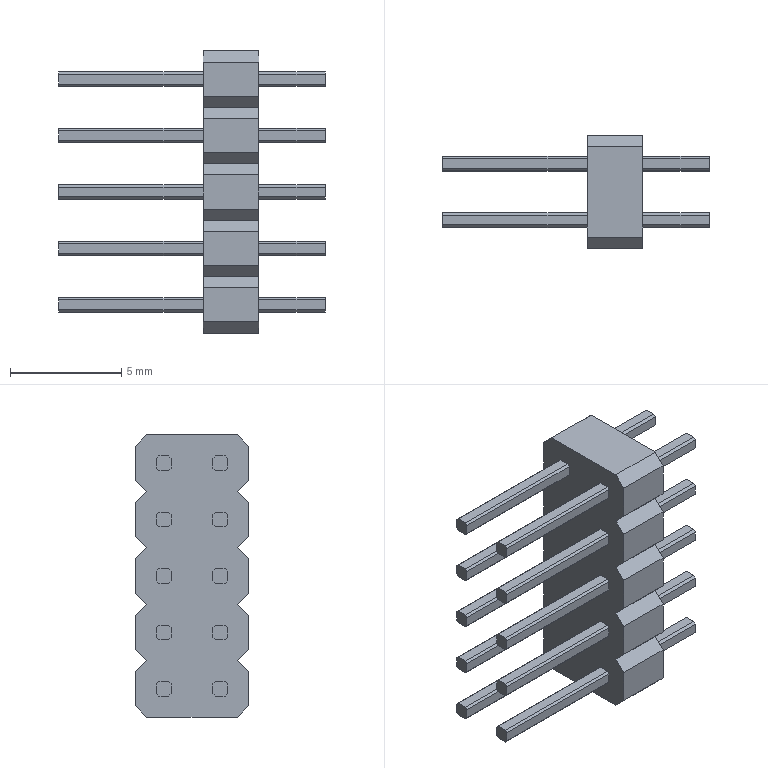Component | SolidWorks | Assembly 1-1_12.Electrical units-2 | 1 solid | 214 faces | box 12 x 5.08 x 12.7 mm | volume 193 mm3 | plane 214
build123d program:
from build123d import *

# Parameters (mm, degrees)
BOSS_EXTRUDE1_DEPTH = 12
LPATTERN1_COUNT     = 2
LPATTERN1_PITCH     = 2.54
BOSS_EXTRUDE2_DEPTH = 2.5
LPATTERN2_COUNT     = 5
LPATTERN2_PITCH     = 2.54


with BuildPart() as part:
    # Sketch1 → Boss-Extrude1 (new body)
    with BuildSketch(Plane(origin=(0, 0, 0), x_dir=(1, 0, 0), z_dir=(0, 1, 0))):
        Polygon((-0.325, -0.225), (-0.225, -0.325), (0.225, -0.325), (0.325, -0.225), (0.325, 0.225), (0.225, 0.325), (-0.225, 0.325), (-0.325, 0.225), align=None)
    extrude(amount=BOSS_EXTRUDE1_DEPTH)


with BuildPart() as lpattern1_1:
    # LPattern1: pattern copy
    add(part.part.moved(Location(Vector(1, 0, 0) * (1 * LPATTERN1_PITCH))))


with BuildPart() as part_1:
    add(part.part)

    add(lpattern1_1.part)  # Boss-Extrude2 merges LPattern1_1
    # Sketch2 → Boss-Extrude2 (add)
    with BuildSketch(Plane(origin=(0, 3, 0), x_dir=(-1, 0, 0), z_dir=(0, -1, 0))):
        Polygon((-3.81, 0.77), (-3.31, 1.27), (0.77, 1.27), (1.27, 0.77), (1.27, -0.77), (0.77, -1.27), (-3.31, -1.27), (-3.81, -0.77), align=None)
    extrude(amount=-BOSS_EXTRUDE2_DEPTH)


with BuildPart() as lpattern2_1:
    # LPattern2: pattern copy
    add(part_1.part.moved(Location(Vector(0, 0, -1) * (1 * LPATTERN2_PITCH))))


with BuildPart() as lpattern2_2:
    # LPattern2: pattern copy
    add(part_1.part.moved(Location(Vector(0, 0, -1) * (2 * LPATTERN2_PITCH))))


with BuildPart() as lpattern2_3:
    # LPattern2: pattern copy
    add(part_1.part.moved(Location(Vector(0, 0, -1) * (3 * LPATTERN2_PITCH))))


with BuildPart() as lpattern2_4:
    # LPattern2: pattern copy
    add(part_1.part.moved(Location(Vector(0, 0, -1) * (4 * LPATTERN2_PITCH))))

    # Combine1: union LPattern2_3, LPattern2_2, LPattern2_1, part
    add(lpattern2_3.part)
    add(lpattern2_2.part)
    add(lpattern2_1.part)
    add(part_1.part)


solid = lpattern2_4.part

# Placed as in the assembly
solid = solid.moved(Location((-15, 10.855, 8.73), (0, 0, 90)))